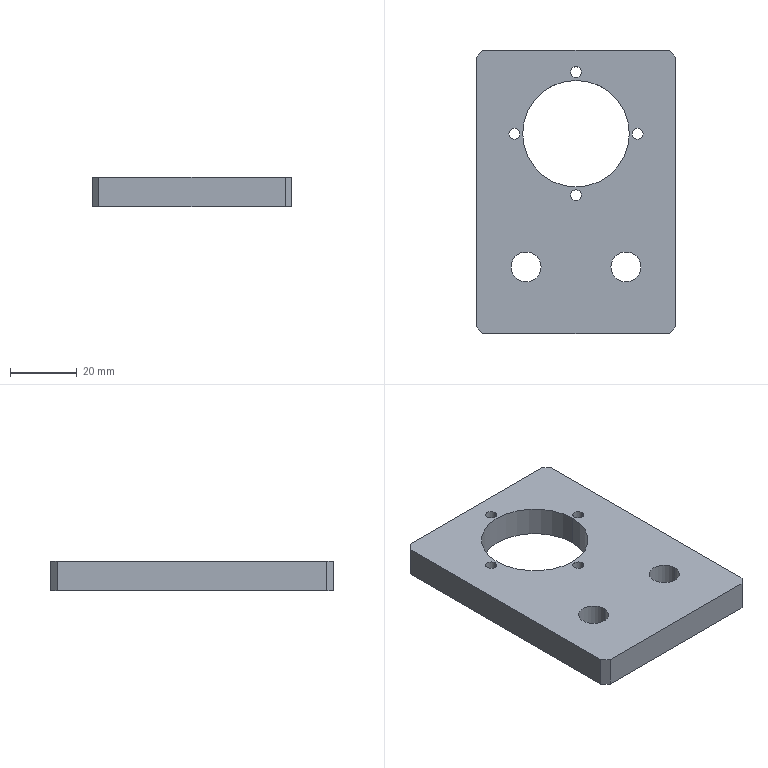Component | SolidWorks | KSD171005A-01-01-19-1 | 1 solid | 24 faces | box 60 x 85 x 9 mm | volume 37137 mm3 | cylinder 14 | plane 10 | commonest cylinder face diameters 3.3 x8 9 x4 32 x2
build123d program:
from build123d import *

# Parameters (mm, degrees)
SKETCH1_W                = 60
SKETCH1_H                = 85
BOSS_EXTRUDE1_DEPTH      = 9
SKETCH2_R                = 16
CUT_EXTRUDE1_DEPTH       = 53.794
F_9_0_9_DIAMETER_HOLE1_D = 9
M4_TAPPED_HOLE1_D        = 3.3
CIRPATTERN1_COUNT        = 4
CHAMFER1_SIZE            = 2


with BuildPart() as part:
    # Sketch1 → Boss-Extrude1 (new body)
    with BuildSketch(Plane.XY):
        Rectangle(SKETCH1_W, SKETCH1_H)
    extrude(amount=BOSS_EXTRUDE1_DEPTH)

    # Sketch2 → Cut-Extrude1 (cut, through all)
    with BuildSketch(Plane.XY.offset(9)):
        with Locations((0, 17.5)):
            Circle(SKETCH2_R)
    extrude(amount=-CUT_EXTRUDE1_DEPTH, mode=Mode.SUBTRACT)

    # 9.0 _9_ Diameter Hole1 (through all)
    with Locations(Plane.XY.offset(9)):
        with Locations((-15, -22.5), (15, -22.5)):
            Hole(F_9_0_9_DIAMETER_HOLE1_D / 2)

    # M4 Tapped Hole1 (through all)
    with Locations(Plane.XY.offset(9)):
        with Locations((0, 36)):
            m4_tapped_hole1 = Hole(M4_TAPPED_HOLE1_D / 2)

    # CirPattern1: M4 Tapped Hole1 ×4 about axis
    cirpattern1_axis = Axis((0, 17.5, 0), (0, 0, 1))
    for i in range(1, CIRPATTERN1_COUNT):
        add(m4_tapped_hole1.rotate(cirpattern1_axis, i * 360 / CIRPATTERN1_COUNT), mode=Mode.SUBTRACT)

    # Chamfer1
    chamfer1_edges = [part.edges().sort_by_distance(p)[0] for p in [
        (30, -42.5, 4.5),
        (-30, -42.5, 4.5),
        (-30, 42.5, 4.5),
        (30, 42.5, 4.5),
    ]]
    chamfer(chamfer1_edges, length=CHAMFER1_SIZE)


solid = part.part

# Placed as in the assembly
solid = solid.moved(Location((-7.111, -1.77, 348), (0, 0, 0)))
STEP:
#1=CARTESIAN_POINT('',(0.3834,0.6193,13.701));
#2=VERTEX_POINT('',#1);
#3=CARTESIAN_POINT('',(0.5133,0.6193,13.701));
#4=VERTEX_POINT('',#3);
#5=CARTESIAN_POINT('',(0.4484,0.6193,13.701));
#6=DIRECTION('',(0.,0.,1.));
#7=DIRECTION('',(1.,0.,0.));
#8=AXIS2_PLACEMENT_3D('',#5,#6,#7);
#9=CIRCLE('',#8,0.06496);
#10=EDGE_CURVE('',#2,#4,#9,.T.);
#11=ORIENTED_EDGE('',*,*,#10,.F.);
#12=CARTESIAN_POINT('',(0.3834,0.6193,14.055));
#13=VERTEX_POINT('',#12);
#14=CARTESIAN_POINT('',(0.3834,0.6193,14.055));
#15=DIRECTION('',(0.,0.,1.));
#16=VECTOR('',#15,39.37);
#17=LINE('',#14,#16);
#18=EDGE_CURVE('',#2,#13,#17,.T.);
#19=ORIENTED_EDGE('',*,*,#18,.T.);
#20=CARTESIAN_POINT('',(0.5133,0.6193,14.055));
#21=VERTEX_POINT('',#20);
#22=CARTESIAN_POINT('',(0.4484,0.6193,14.055));
#23=DIRECTION('',(0.,0.,1.));
#24=DIRECTION('',(1.,0.,0.));
#25=AXIS2_PLACEMENT_3D('',#22,#23,#24);
#26=CIRCLE('',#25,0.06496);
#27=EDGE_CURVE('',#13,#21,#26,.T.);
#28=ORIENTED_EDGE('',*,*,#27,.T.);
#29=CARTESIAN_POINT('',(0.5133,0.6193,14.055));
#30=DIRECTION('',(0.,0.,1.));
#31=VECTOR('',#30,39.37);
#32=LINE('',#29,#31);
#33=EDGE_CURVE('',#4,#21,#32,.T.);
#34=ORIENTED_EDGE('',*,*,#33,.F.);
#35=EDGE_LOOP('',(#11,#19,#28,#34));
#36=FACE_OUTER_BOUND('',#35,.T.);
#37=CARTESIAN_POINT('',(0.4484,0.6193,14.055));
#38=DIRECTION('',(0.,0.,1.));
#39=DIRECTION('',(1.,0.,0.));
#40=AXIS2_PLACEMENT_3D('',#37,#38,#39);
#41=CYLINDRICAL_SURFACE('',#40,0.06496);
#42=ADVANCED_FACE('',(#36),#41,.F.);
#43=CARTESIAN_POINT('',(-0.3449,-0.1091,13.701));
#44=VERTEX_POINT('',#43);
#45=CARTESIAN_POINT('',(-0.215,-0.1091,13.701));
#46=VERTEX_POINT('',#45);
#47=CARTESIAN_POINT('',(-0.28,-0.1091,13.701));
#48=DIRECTION('',(0.,0.,1.));
#49=DIRECTION('',(1.,0.,0.));
#50=AXIS2_PLACEMENT_3D('',#47,#48,#49);
#51=CIRCLE('',#50,0.06496);
#52=EDGE_CURVE('',#44,#46,#51,.T.);
#53=ORIENTED_EDGE('',*,*,#52,.F.);
#54=CARTESIAN_POINT('',(-0.3449,-0.1091,14.055));
#55=VERTEX_POINT('',#54);
#56=CARTESIAN_POINT('',(-0.3449,-0.1091,14.055));
#57=DIRECTION('',(0.,0.,1.));
#58=VECTOR('',#57,39.37);
#59=LINE('',#56,#58);
#60=EDGE_CURVE('',#44,#55,#59,.T.);
#61=ORIENTED_EDGE('',*,*,#60,.T.);
#62=CARTESIAN_POINT('',(-0.215,-0.1091,14.055));
#63=VERTEX_POINT('',#62);
#64=CARTESIAN_POINT('',(-0.28,-0.1091,14.055));
#65=DIRECTION('',(0.,0.,1.));
#66=DIRECTION('',(1.,0.,0.));
#67=AXIS2_PLACEMENT_3D('',#64,#65,#66);
#68=CIRCLE('',#67,0.06496);
#69=EDGE_CURVE('',#55,#63,#68,.T.);
#70=ORIENTED_EDGE('',*,*,#69,.T.);
#71=CARTESIAN_POINT('',(-0.215,-0.1091,14.055));
#72=DIRECTION('',(0.,0.,1.));
#73=VECTOR('',#72,39.37);
#74=LINE('',#71,#73);
#75=EDGE_CURVE('',#46,#63,#74,.T.);
#76=ORIENTED_EDGE('',*,*,#75,.F.);
#77=EDGE_LOOP('',(#53,#61,#70,#76));
#78=FACE_OUTER_BOUND('',#77,.T.);
#79=CARTESIAN_POINT('',(-0.28,-0.1091,14.055));
#80=DIRECTION('',(0.,0.,1.));
#81=DIRECTION('',(1.,0.,0.));
#82=AXIS2_PLACEMENT_3D('',#79,#80,#81);
#83=CYLINDRICAL_SURFACE('',#82,0.06496);
#84=ADVANCED_FACE('',(#78),#83,.F.);
#85=CARTESIAN_POINT('',(-1.073,0.6193,13.701));
#86=VERTEX_POINT('',#85);
#87=CARTESIAN_POINT('',(-0.9434,0.6193,13.701));
#88=VERTEX_POINT('',#87);
#89=CARTESIAN_POINT('',(-1.008,0.6193,13.701));
#90=DIRECTION('',(0.,0.,1.));
#91=DIRECTION('',(1.,0.,0.));
#92=AXIS2_PLACEMENT_3D('',#89,#90,#91);
#93=CIRCLE('',#92,0.06496);
#94=EDGE_CURVE('',#86,#88,#93,.T.);
#95=ORIENTED_EDGE('',*,*,#94,.F.);
#96=CARTESIAN_POINT('',(-1.073,0.6193,14.055));
#97=VERTEX_POINT('',#96);
#98=CARTESIAN_POINT('',(-1.073,0.6193,14.055));
#99=DIRECTION('',(0.,0.,1.));
#100=VECTOR('',#99,39.37);
#101=LINE('',#98,#100);
#102=EDGE_CURVE('',#86,#97,#101,.T.);
#103=ORIENTED_EDGE('',*,*,#102,.T.);
#104=CARTESIAN_POINT('',(-0.9434,0.6193,14.055));
#105=VERTEX_POINT('',#104);
#106=CARTESIAN_POINT('',(-1.008,0.6193,14.055));
#107=DIRECTION('',(0.,0.,1.));
#108=DIRECTION('',(1.,0.,0.));
#109=AXIS2_PLACEMENT_3D('',#106,#107,#108);
#110=CIRCLE('',#109,0.06496);
#111=EDGE_CURVE('',#97,#105,#110,.T.);
#112=ORIENTED_EDGE('',*,*,#111,.T.);
#113=CARTESIAN_POINT('',(-0.9434,0.6193,14.055));
#114=DIRECTION('',(0.,0.,1.));
#115=VECTOR('',#114,39.37);
#116=LINE('',#113,#115);
#117=EDGE_CURVE('',#88,#105,#116,.T.);
#118=ORIENTED_EDGE('',*,*,#117,.F.);
#119=EDGE_LOOP('',(#95,#103,#112,#118));
#120=FACE_OUTER_BOUND('',#119,.T.);
#121=CARTESIAN_POINT('',(-1.008,0.6193,14.055));
#122=DIRECTION('',(0.,0.,1.));
#123=DIRECTION('',(1.,0.,0.));
#124=AXIS2_PLACEMENT_3D('',#121,#122,#123);
#125=CYLINDRICAL_SURFACE('',#124,0.06496);
#126=ADVANCED_FACE('',(#120),#125,.F.);
#127=CARTESIAN_POINT('',(-0.3449,1.348,13.701));
#128=VERTEX_POINT('',#127);
#129=CARTESIAN_POINT('',(-0.215,1.348,13.701));
#130=VERTEX_POINT('',#129);
#131=CARTESIAN_POINT('',(-0.28,1.348,13.701));
#132=DIRECTION('',(0.,0.,1.));
#133=DIRECTION('',(1.,0.,0.));
#134=AXIS2_PLACEMENT_3D('',#131,#132,#133);
#135=CIRCLE('',#134,0.06496);
#136=EDGE_CURVE('',#128,#130,#135,.T.);
#137=ORIENTED_EDGE('',*,*,#136,.F.);
#138=CARTESIAN_POINT('',(-0.3449,1.348,14.055));
#139=VERTEX_POINT('',#138);
#140=CARTESIAN_POINT('',(-0.3449,1.348,14.055));
#141=DIRECTION('',(0.,0.,1.));
#142=VECTOR('',#141,39.37);
#143=LINE('',#140,#142);
#144=EDGE_CURVE('',#128,#139,#143,.T.);
#145=ORIENTED_EDGE('',*,*,#144,.T.);
#146=CARTESIAN_POINT('',(-0.215,1.348,14.055));
#147=VERTEX_POINT('',#146);
#148=CARTESIAN_POINT('',(-0.28,1.348,14.055));
#149=DIRECTION('',(0.,0.,1.));
#150=DIRECTION('',(1.,0.,0.));
#151=AXIS2_PLACEMENT_3D('',#148,#149,#150);
#152=CIRCLE('',#151,0.06496);
#153=EDGE_CURVE('',#139,#147,#152,.T.);
#154=ORIENTED_EDGE('',*,*,#153,.T.);
#155=CARTESIAN_POINT('',(-0.215,1.348,14.055));
#156=DIRECTION('',(0.,0.,1.));
#157=VECTOR('',#156,39.37);
#158=LINE('',#155,#157);
#159=EDGE_CURVE('',#130,#147,#158,.T.);
#160=ORIENTED_EDGE('',*,*,#159,.F.);
#161=EDGE_LOOP('',(#137,#145,#154,#160));
#162=FACE_OUTER_BOUND('',#161,.T.);
#163=CARTESIAN_POINT('',(-0.28,1.348,14.055));
#164=DIRECTION('',(0.,0.,1.));
#165=DIRECTION('',(1.,0.,0.));
#166=AXIS2_PLACEMENT_3D('',#163,#164,#165);
#167=CYLINDRICAL_SURFACE('',#166,0.06496);
#168=ADVANCED_FACE('',(#162),#167,.F.);
#169=CARTESIAN_POINT('',(-1.048,-0.9555,13.701));
#170=VERTEX_POINT('',#169);
#171=CARTESIAN_POINT('',(-0.6934,-0.9555,13.701));
#172=VERTEX_POINT('',#171);
#173=CARTESIAN_POINT('',(-0.8705,-0.9555,13.701));
#174=DIRECTION('',(0.,0.,1.));
#175=DIRECTION('',(1.,0.,0.));
#176=AXIS2_PLACEMENT_3D('',#173,#174,#175);
#177=CIRCLE('',#176,0.1772);
#178=EDGE_CURVE('',#170,#172,#177,.T.);
#179=ORIENTED_EDGE('',*,*,#178,.F.);
#180=CARTESIAN_POINT('',(-1.048,-0.9555,14.055));
#181=VERTEX_POINT('',#180);
#182=CARTESIAN_POINT('',(-1.048,-0.9555,14.055));
#183=DIRECTION('',(0.,0.,1.));
#184=VECTOR('',#183,39.37);
#185=LINE('',#182,#184);
#186=EDGE_CURVE('',#170,#181,#185,.T.);
#187=ORIENTED_EDGE('',*,*,#186,.T.);
#188=CARTESIAN_POINT('',(-0.6934,-0.9555,14.055));
#189=VERTEX_POINT('',#188);
#190=CARTESIAN_POINT('',(-0.8705,-0.9555,14.055));
#191=DIRECTION('',(0.,0.,1.));
#192=DIRECTION('',(1.,0.,0.));
#193=AXIS2_PLACEMENT_3D('',#190,#191,#192);
#194=CIRCLE('',#193,0.1772);
#195=EDGE_CURVE('',#181,#189,#194,.T.);
#196=ORIENTED_EDGE('',*,*,#195,.T.);
#197=CARTESIAN_POINT('',(-0.6934,-0.9555,14.055));
#198=DIRECTION('',(0.,0.,1.));
#199=VECTOR('',#198,39.37);
#200=LINE('',#197,#199);
#201=EDGE_CURVE('',#172,#189,#200,.T.);
#202=ORIENTED_EDGE('',*,*,#201,.F.);
#203=EDGE_LOOP('',(#179,#187,#196,#202));
#204=FACE_OUTER_BOUND('',#203,.T.);
#205=CARTESIAN_POINT('',(-0.8705,-0.9555,14.055));
#206=DIRECTION('',(0.,0.,1.));
#207=DIRECTION('',(1.,0.,0.));
#208=AXIS2_PLACEMENT_3D('',#205,#206,#207);
#209=CYLINDRICAL_SURFACE('',#208,0.1772);
#210=ADVANCED_FACE('',(#204),#209,.F.);
#211=CARTESIAN_POINT('',(0.1334,-0.9555,13.701));
#212=VERTEX_POINT('',#211);
#213=CARTESIAN_POINT('',(0.4877,-0.9555,13.701));
#214=VERTEX_POINT('',#213);
#215=CARTESIAN_POINT('',(0.3106,-0.9555,13.701));
#216=DIRECTION('',(0.,0.,1.));
#217=DIRECTION('',(1.,0.,0.));
#218=AXIS2_PLACEMENT_3D('',#215,#216,#217);
#219=CIRCLE('',#218,0.1772);
#220=EDGE_CURVE('',#212,#214,#219,.T.);
#221=ORIENTED_EDGE('',*,*,#220,.F.);
#222=CARTESIAN_POINT('',(0.1334,-0.9555,14.055));
#223=VERTEX_POINT('',#222);
#224=CARTESIAN_POINT('',(0.1334,-0.9555,14.055));
#225=DIRECTION('',(0.,0.,1.));
#226=VECTOR('',#225,39.37);
#227=LINE('',#224,#226);
#228=EDGE_CURVE('',#212,#223,#227,.T.);
#229=ORIENTED_EDGE('',*,*,#228,.T.);
#230=CARTESIAN_POINT('',(0.4877,-0.9555,14.055));
#231=VERTEX_POINT('',#230);
#232=CARTESIAN_POINT('',(0.3106,-0.9555,14.055));
#233=DIRECTION('',(0.,0.,1.));
#234=DIRECTION('',(1.,0.,0.));
#235=AXIS2_PLACEMENT_3D('',#232,#233,#234);
#236=CIRCLE('',#235,0.1772);
#237=EDGE_CURVE('',#223,#231,#236,.T.);
#238=ORIENTED_EDGE('',*,*,#237,.T.);
#239=CARTESIAN_POINT('',(0.4877,-0.9555,14.055));
#240=DIRECTION('',(0.,0.,1.));
#241=VECTOR('',#240,39.37);
#242=LINE('',#239,#241);
#243=EDGE_CURVE('',#214,#231,#242,.T.);
#244=ORIENTED_EDGE('',*,*,#243,.F.);
#245=EDGE_LOOP('',(#221,#229,#238,#244));
#246=FACE_OUTER_BOUND('',#245,.T.);
#247=CARTESIAN_POINT('',(0.3106,-0.9555,14.055));
#248=DIRECTION('',(0.,0.,1.));
#249=DIRECTION('',(1.,0.,0.));
#250=AXIS2_PLACEMENT_3D('',#247,#248,#249);
#251=CYLINDRICAL_SURFACE('',#250,0.1772);
#252=ADVANCED_FACE('',(#246),#251,.F.);
#253=CARTESIAN_POINT('',(-0.9099,0.6193,13.701));
#254=VERTEX_POINT('',#253);
#255=CARTESIAN_POINT('',(0.3499,0.6193,13.701));
#256=VERTEX_POINT('',#255);
#257=CARTESIAN_POINT('',(-0.28,0.6193,13.701));
#258=DIRECTION('',(0.,0.,1.));
#259=DIRECTION('',(1.,0.,0.));
#260=AXIS2_PLACEMENT_3D('',#257,#258,#259);
#261=CIRCLE('',#260,0.6299);
#262=EDGE_CURVE('',#254,#256,#261,.T.);
#263=ORIENTED_EDGE('',*,*,#262,.F.);
#264=CARTESIAN_POINT('',(-0.9099,0.6193,14.055));
#265=VERTEX_POINT('',#264);
#266=CARTESIAN_POINT('',(-0.9099,0.6193,13.701));
#267=DIRECTION('',(0.,0.,1.));
#268=VECTOR('',#267,39.37);
#269=LINE('',#266,#268);
#270=EDGE_CURVE('',#254,#265,#269,.T.);
#271=ORIENTED_EDGE('',*,*,#270,.T.);
#272=CARTESIAN_POINT('',(0.3499,0.6193,14.055));
#273=VERTEX_POINT('',#272);
#274=CARTESIAN_POINT('',(-0.28,0.6193,14.055));
#275=DIRECTION('',(0.,0.,1.));
#276=DIRECTION('',(1.,0.,0.));
#277=AXIS2_PLACEMENT_3D('',#274,#275,#276);
#278=CIRCLE('',#277,0.6299);
#279=EDGE_CURVE('',#265,#273,#278,.T.);
#280=ORIENTED_EDGE('',*,*,#279,.T.);
#281=CARTESIAN_POINT('',(0.3499,0.6193,13.701));
#282=DIRECTION('',(0.,0.,1.));
#283=VECTOR('',#282,39.37);
#284=LINE('',#281,#283);
#285=EDGE_CURVE('',#256,#273,#284,.T.);
#286=ORIENTED_EDGE('',*,*,#285,.F.);
#287=EDGE_LOOP('',(#263,#271,#280,#286));
#288=FACE_OUTER_BOUND('',#287,.T.);
#289=CARTESIAN_POINT('',(-0.28,0.6193,13.701));
#290=DIRECTION('',(0.,0.,1.));
#291=DIRECTION('',(1.,0.,0.));
#292=AXIS2_PLACEMENT_3D('',#289,#290,#291);
#293=CYLINDRICAL_SURFACE('',#292,0.6299);
#294=ADVANCED_FACE('',(#288),#293,.F.);
#295=CARTESIAN_POINT('',(0.9011,-1.664,13.701));
#296=VERTEX_POINT('',#295);
#297=CARTESIAN_POINT('',(0.9011,1.525,13.701));
#298=VERTEX_POINT('',#297);
#299=CARTESIAN_POINT('',(0.9011,1.604,13.701));
#300=DIRECTION('',(-0.,1.,0.));
#301=VECTOR('',#300,39.37);
#302=LINE('',#299,#301);
#303=EDGE_CURVE('',#296,#298,#302,.T.);
#304=ORIENTED_EDGE('',*,*,#303,.T.);
#305=CARTESIAN_POINT('',(0.9011,1.525,14.055));
#306=VERTEX_POINT('',#305);
#307=CARTESIAN_POINT('',(0.9011,1.525,14.055));
#308=DIRECTION('',(0.,0.,1.));
#309=VECTOR('',#308,39.37);
#310=LINE('',#307,#309);
#311=EDGE_CURVE('',#298,#306,#310,.T.);
#312=ORIENTED_EDGE('',*,*,#311,.T.);
#313=CARTESIAN_POINT('',(0.9011,-1.664,14.055));
#314=VERTEX_POINT('',#313);
#315=CARTESIAN_POINT('',(0.9011,1.604,14.055));
#316=DIRECTION('',(-0.,1.,0.));
#317=VECTOR('',#316,39.37);
#318=LINE('',#315,#317);
#319=EDGE_CURVE('',#314,#306,#318,.T.);
#320=ORIENTED_EDGE('',*,*,#319,.F.);
#321=CARTESIAN_POINT('',(0.9011,-1.664,14.055));
#322=DIRECTION('',(0.,0.,-1.));
#323=VECTOR('',#322,39.37);
#324=LINE('',#321,#323);
#325=EDGE_CURVE('',#314,#296,#324,.T.);
#326=ORIENTED_EDGE('',*,*,#325,.T.);
#327=EDGE_LOOP('',(#304,#312,#320,#326));
#328=FACE_OUTER_BOUND('',#327,.T.);
#329=CARTESIAN_POINT('',(0.9011,1.604,14.055));
#330=DIRECTION('',(-1.,-0.,0.));
#331=DIRECTION('',(0.,-1.,0.));
#332=AXIS2_PLACEMENT_3D('',#329,#330,#331);
#333=PLANE('',#332);
#334=ADVANCED_FACE('',(#328),#333,.F.);
#335=CARTESIAN_POINT('',(0.8224,1.604,13.701));
#336=VERTEX_POINT('',#335);
#337=CARTESIAN_POINT('',(-1.382,1.604,13.701));
#338=VERTEX_POINT('',#337);
#339=CARTESIAN_POINT('',(-1.461,1.604,13.701));
#340=DIRECTION('',(-1.,0.,0.));
#341=VECTOR('',#340,39.37);
#342=LINE('',#339,#341);
#343=EDGE_CURVE('',#336,#338,#342,.T.);
#344=ORIENTED_EDGE('',*,*,#343,.T.);
#345=CARTESIAN_POINT('',(-1.382,1.604,14.055));
#346=VERTEX_POINT('',#345);
#347=CARTESIAN_POINT('',(-1.382,1.604,14.055));
#348=DIRECTION('',(0.,0.,1.));
#349=VECTOR('',#348,39.37);
#350=LINE('',#347,#349);
#351=EDGE_CURVE('',#338,#346,#350,.T.);
#352=ORIENTED_EDGE('',*,*,#351,.T.);
#353=CARTESIAN_POINT('',(0.8224,1.604,14.055));
#354=VERTEX_POINT('',#353);
#355=CARTESIAN_POINT('',(-1.461,1.604,14.055));
#356=DIRECTION('',(-1.,0.,0.));
#357=VECTOR('',#356,39.37);
#358=LINE('',#355,#357);
#359=EDGE_CURVE('',#354,#346,#358,.T.);
#360=ORIENTED_EDGE('',*,*,#359,.F.);
#361=CARTESIAN_POINT('',(0.8224,1.604,14.055));
#362=DIRECTION('',(0.,0.,-1.));
#363=VECTOR('',#362,39.37);
#364=LINE('',#361,#363);
#365=EDGE_CURVE('',#354,#336,#364,.T.);
#366=ORIENTED_EDGE('',*,*,#365,.T.);
#367=EDGE_LOOP('',(#344,#352,#360,#366));
#368=FACE_OUTER_BOUND('',#367,.T.);
#369=CARTESIAN_POINT('',(-1.461,1.604,14.055));
#370=DIRECTION('',(0.,-1.,0.));
#371=DIRECTION('',(0.,0.,-1.));
#372=AXIS2_PLACEMENT_3D('',#369,#370,#371);
#373=PLANE('',#372);
#374=ADVANCED_FACE('',(#368),#373,.F.);
#375=CARTESIAN_POINT('',(-1.461,1.525,14.055));
#376=VERTEX_POINT('',#375);
#377=CARTESIAN_POINT('',(-1.461,-1.664,14.055));
#378=VERTEX_POINT('',#377);
#379=CARTESIAN_POINT('',(-1.461,1.604,14.055));
#380=DIRECTION('',(0.,-1.,0.));
#381=VECTOR('',#380,39.37);
#382=LINE('',#379,#381);
#383=EDGE_CURVE('',#376,#378,#382,.T.);
#384=ORIENTED_EDGE('',*,*,#383,.F.);
#385=CARTESIAN_POINT('',(-1.461,1.525,13.701));
#386=VERTEX_POINT('',#385);
#387=CARTESIAN_POINT('',(-1.461,1.525,14.055));
#388=DIRECTION('',(0.,0.,-1.));
#389=VECTOR('',#388,39.37);
#390=LINE('',#387,#389);
#391=EDGE_CURVE('',#376,#386,#390,.T.);
#392=ORIENTED_EDGE('',*,*,#391,.T.);
#393=CARTESIAN_POINT('',(-1.461,-1.664,13.701));
#394=VERTEX_POINT('',#393);
#395=CARTESIAN_POINT('',(-1.461,1.604,13.701));
#396=DIRECTION('',(0.,-1.,0.));
#397=VECTOR('',#396,39.37);
#398=LINE('',#395,#397);
#399=EDGE_CURVE('',#386,#394,#398,.T.);
#400=ORIENTED_EDGE('',*,*,#399,.T.);
#401=CARTESIAN_POINT('',(-1.461,-1.664,14.055));
#402=DIRECTION('',(0.,0.,1.));
#403=VECTOR('',#402,39.37);
#404=LINE('',#401,#403);
#405=EDGE_CURVE('',#394,#378,#404,.T.);
#406=ORIENTED_EDGE('',*,*,#405,.T.);
#407=EDGE_LOOP('',(#384,#392,#400,#406));
#408=FACE_OUTER_BOUND('',#407,.T.);
#409=CARTESIAN_POINT('',(-1.461,1.604,14.055));
#410=DIRECTION('',(1.,0.,0.));
#411=DIRECTION('',(-0.,1.,0.));
#412=AXIS2_PLACEMENT_3D('',#409,#410,#411);
#413=PLANE('',#412);
#414=ADVANCED_FACE('',(#408),#413,.F.);
#415=CARTESIAN_POINT('',(-1.382,-1.743,13.701));
#416=VERTEX_POINT('',#415);
#417=CARTESIAN_POINT('',(0.8224,-1.743,13.701));
#418=VERTEX_POINT('',#417);
#419=CARTESIAN_POINT('',(-1.461,-1.743,13.701));
#420=DIRECTION('',(1.,0.,0.));
#421=VECTOR('',#420,39.37);
#422=LINE('',#419,#421);
#423=EDGE_CURVE('',#416,#418,#422,.T.);
#424=ORIENTED_EDGE('',*,*,#423,.T.);
#425=CARTESIAN_POINT('',(0.8224,-1.743,14.055));
#426=VERTEX_POINT('',#425);
#427=CARTESIAN_POINT('',(0.8224,-1.743,14.055));
#428=DIRECTION('',(0.,0.,1.));
#429=VECTOR('',#428,39.37);
#430=LINE('',#427,#429);
#431=EDGE_CURVE('',#418,#426,#430,.T.);
#432=ORIENTED_EDGE('',*,*,#431,.T.);
#433=CARTESIAN_POINT('',(-1.382,-1.743,14.055));
#434=VERTEX_POINT('',#433);
#435=CARTESIAN_POINT('',(-1.461,-1.743,14.055));
#436=DIRECTION('',(1.,0.,0.));
#437=VECTOR('',#436,39.37);
#438=LINE('',#435,#437);
#439=EDGE_CURVE('',#434,#426,#438,.T.);
#440=ORIENTED_EDGE('',*,*,#439,.F.);
#441=CARTESIAN_POINT('',(-1.382,-1.743,14.055));
#442=DIRECTION('',(0.,0.,-1.));
#443=VECTOR('',#442,39.37);
#444=LINE('',#441,#443);
#445=EDGE_CURVE('',#434,#416,#444,.T.);
#446=ORIENTED_EDGE('',*,*,#445,.T.);
#447=EDGE_LOOP('',(#424,#432,#440,#446));
#448=FACE_OUTER_BOUND('',#447,.T.);
#449=CARTESIAN_POINT('',(-1.461,-1.743,14.055));
#450=DIRECTION('',(0.,1.,0.));
#451=DIRECTION('',(0.,0.,1.));
#452=AXIS2_PLACEMENT_3D('',#449,#450,#451);
#453=PLANE('',#452);
#454=ADVANCED_FACE('',(#448),#453,.F.);
#455=CARTESIAN_POINT('',(0.4484,0.6193,14.055));
#456=DIRECTION('',(0.,0.,1.));
#457=DIRECTION('',(1.,0.,0.));
#458=AXIS2_PLACEMENT_3D('',#455,#456,#457);
#459=CIRCLE('',#458,0.06496);
#460=EDGE_CURVE('',#21,#13,#459,.T.);
#461=ORIENTED_EDGE('',*,*,#460,.F.);
#462=ORIENTED_EDGE('',*,*,#27,.F.);
#463=EDGE_LOOP('',(#461,#462));
#464=FACE_BOUND('',#463,.T.);
#465=CARTESIAN_POINT('',(-0.28,-0.1091,14.055));
#466=DIRECTION('',(0.,0.,1.));
#467=DIRECTION('',(1.,0.,0.));
#468=AXIS2_PLACEMENT_3D('',#465,#466,#467);
#469=CIRCLE('',#468,0.06496);
#470=EDGE_CURVE('',#63,#55,#469,.T.);
#471=ORIENTED_EDGE('',*,*,#470,.F.);
#472=ORIENTED_EDGE('',*,*,#69,.F.);
#473=EDGE_LOOP('',(#471,#472));
#474=FACE_BOUND('',#473,.T.);
#475=CARTESIAN_POINT('',(-1.008,0.6193,14.055));
#476=DIRECTION('',(0.,0.,1.));
#477=DIRECTION('',(1.,0.,0.));
#478=AXIS2_PLACEMENT_3D('',#475,#476,#477);
#479=CIRCLE('',#478,0.06496);
#480=EDGE_CURVE('',#105,#97,#479,.T.);
#481=ORIENTED_EDGE('',*,*,#480,.F.);
#482=ORIENTED_EDGE('',*,*,#111,.F.);
#483=EDGE_LOOP('',(#481,#482));
#484=FACE_BOUND('',#483,.T.);
#485=CARTESIAN_POINT('',(-0.28,1.348,14.055));
#486=DIRECTION('',(0.,0.,1.));
#487=DIRECTION('',(1.,0.,0.));
#488=AXIS2_PLACEMENT_3D('',#485,#486,#487);
#489=CIRCLE('',#488,0.06496);
#490=EDGE_CURVE('',#147,#139,#489,.T.);
#491=ORIENTED_EDGE('',*,*,#490,.F.);
#492=ORIENTED_EDGE('',*,*,#153,.F.);
#493=EDGE_LOOP('',(#491,#492));
#494=FACE_BOUND('',#493,.T.);
#495=CARTESIAN_POINT('',(-0.8705,-0.9555,14.055));
#496=DIRECTION('',(0.,0.,1.));
#497=DIRECTION('',(1.,0.,0.));
#498=AXIS2_PLACEMENT_3D('',#495,#496,#497);
#499=CIRCLE('',#498,0.1772);
#500=EDGE_CURVE('',#189,#181,#499,.T.);
#501=ORIENTED_EDGE('',*,*,#500,.F.);
#502=ORIENTED_EDGE('',*,*,#195,.F.);
#503=EDGE_LOOP('',(#501,#502));
#504=FACE_BOUND('',#503,.T.);
#505=CARTESIAN_POINT('',(0.3106,-0.9555,14.055));
#506=DIRECTION('',(0.,0.,1.));
#507=DIRECTION('',(1.,0.,0.));
#508=AXIS2_PLACEMENT_3D('',#505,#506,#507);
#509=CIRCLE('',#508,0.1772);
#510=EDGE_CURVE('',#231,#223,#509,.T.);
#511=ORIENTED_EDGE('',*,*,#510,.F.);
#512=ORIENTED_EDGE('',*,*,#237,.F.);
#513=EDGE_LOOP('',(#511,#512));
#514=FACE_BOUND('',#513,.T.);
#515=CARTESIAN_POINT('',(-0.28,0.6193,14.055));
#516=DIRECTION('',(0.,0.,1.));
#517=DIRECTION('',(1.,0.,0.));
#518=AXIS2_PLACEMENT_3D('',#515,#516,#517);
#519=CIRCLE('',#518,0.6299);
#520=EDGE_CURVE('',#273,#265,#519,.T.);
#521=ORIENTED_EDGE('',*,*,#520,.F.);
#522=ORIENTED_EDGE('',*,*,#279,.F.);
#523=EDGE_LOOP('',(#521,#522));
#524=FACE_BOUND('',#523,.T.);
#525=ORIENTED_EDGE('',*,*,#359,.T.);
#526=CARTESIAN_POINT('',(-1.668,1.318,14.055));
#527=DIRECTION('',(-0.7071,-0.7071,0.));
#528=VECTOR('',#527,39.37);
#529=LINE('',#526,#528);
#530=EDGE_CURVE('',#346,#376,#529,.T.);
#531=ORIENTED_EDGE('',*,*,#530,.T.);
#532=ORIENTED_EDGE('',*,*,#383,.T.);
#533=CARTESIAN_POINT('',(-1.668,-1.457,14.055));
#534=DIRECTION('',(0.7071,-0.7071,0.));
#535=VECTOR('',#534,39.37);
#536=LINE('',#533,#535);
#537=EDGE_CURVE('',#378,#434,#536,.T.);
#538=ORIENTED_EDGE('',*,*,#537,.T.);
#539=ORIENTED_EDGE('',*,*,#439,.T.);
#540=CARTESIAN_POINT('',(1.108,-1.457,14.055));
#541=DIRECTION('',(0.7071,0.7071,0.));
#542=VECTOR('',#541,39.37);
#543=LINE('',#540,#542);
#544=EDGE_CURVE('',#426,#314,#543,.T.);
#545=ORIENTED_EDGE('',*,*,#544,.T.);
#546=ORIENTED_EDGE('',*,*,#319,.T.);
#547=CARTESIAN_POINT('',(1.108,1.318,14.055));
#548=DIRECTION('',(-0.7071,0.7071,0.));
#549=VECTOR('',#548,39.37);
#550=LINE('',#547,#549);
#551=EDGE_CURVE('',#306,#354,#550,.T.);
#552=ORIENTED_EDGE('',*,*,#551,.T.);
#553=EDGE_LOOP('',(#525,#531,#532,#538,#539,#545,#546,#552));
#554=FACE_OUTER_BOUND('',#553,.T.);
#555=CARTESIAN_POINT('',(-0.28,-0.0697,14.055));
#556=DIRECTION('',(0.,0.,1.));
#557=DIRECTION('',(1.,0.,0.));
#558=AXIS2_PLACEMENT_3D('',#555,#556,#557);
#559=PLANE('',#558);
#560=ADVANCED_FACE('',(#464,#474,#484,#494,#504,#514,#524,#554),#559,.T.);
#561=CARTESIAN_POINT('',(0.4484,0.6193,13.701));
#562=DIRECTION('',(0.,0.,1.));
#563=DIRECTION('',(1.,0.,0.));
#564=AXIS2_PLACEMENT_3D('',#561,#562,#563);
#565=CIRCLE('',#564,0.06496);
#566=EDGE_CURVE('',#4,#2,#565,.T.);
#567=ORIENTED_EDGE('',*,*,#566,.T.);
#568=ORIENTED_EDGE('',*,*,#10,.T.);
#569=EDGE_LOOP('',(#567,#568));
#570=FACE_BOUND('',#569,.T.);
#571=CARTESIAN_POINT('',(-0.28,-0.1091,13.701));
#572=DIRECTION('',(0.,0.,1.));
#573=DIRECTION('',(1.,0.,0.));
#574=AXIS2_PLACEMENT_3D('',#571,#572,#573);
#575=CIRCLE('',#574,0.06496);
#576=EDGE_CURVE('',#46,#44,#575,.T.);
#577=ORIENTED_EDGE('',*,*,#576,.T.);
#578=ORIENTED_EDGE('',*,*,#52,.T.);
#579=EDGE_LOOP('',(#577,#578));
#580=FACE_BOUND('',#579,.T.);
#581=CARTESIAN_POINT('',(-1.008,0.6193,13.701));
#582=DIRECTION('',(0.,0.,1.));
#583=DIRECTION('',(1.,0.,0.));
#584=AXIS2_PLACEMENT_3D('',#581,#582,#583);
#585=CIRCLE('',#584,0.06496);
#586=EDGE_CURVE('',#88,#86,#585,.T.);
#587=ORIENTED_EDGE('',*,*,#586,.T.);
#588=ORIENTED_EDGE('',*,*,#94,.T.);
#589=EDGE_LOOP('',(#587,#588));
#590=FACE_BOUND('',#589,.T.);
#591=CARTESIAN_POINT('',(-0.28,1.348,13.701));
#592=DIRECTION('',(0.,0.,1.));
#593=DIRECTION('',(1.,0.,0.));
#594=AXIS2_PLACEMENT_3D('',#591,#592,#593);
#595=CIRCLE('',#594,0.06496);
#596=EDGE_CURVE('',#130,#128,#595,.T.);
#597=ORIENTED_EDGE('',*,*,#596,.T.);
#598=ORIENTED_EDGE('',*,*,#136,.T.);
#599=EDGE_LOOP('',(#597,#598));
#600=FACE_BOUND('',#599,.T.);
#601=CARTESIAN_POINT('',(-0.8705,-0.9555,13.701));
#602=DIRECTION('',(0.,0.,1.));
#603=DIRECTION('',(1.,0.,0.));
#604=AXIS2_PLACEMENT_3D('',#601,#602,#603);
#605=CIRCLE('',#604,0.1772);
#606=EDGE_CURVE('',#172,#170,#605,.T.);
#607=ORIENTED_EDGE('',*,*,#606,.T.);
#608=ORIENTED_EDGE('',*,*,#178,.T.);
#609=EDGE_LOOP('',(#607,#608));
#610=FACE_BOUND('',#609,.T.);
#611=CARTESIAN_POINT('',(0.3106,-0.9555,13.701));
#612=DIRECTION('',(0.,0.,1.));
#613=DIRECTION('',(1.,0.,0.));
#614=AXIS2_PLACEMENT_3D('',#611,#612,#613);
#615=CIRCLE('',#614,0.1772);
#616=EDGE_CURVE('',#214,#212,#615,.T.);
#617=ORIENTED_EDGE('',*,*,#616,.T.);
#618=ORIENTED_EDGE('',*,*,#220,.T.);
#619=EDGE_LOOP('',(#617,#618));
#620=FACE_BOUND('',#619,.T.);
#621=CARTESIAN_POINT('',(-0.28,0.6193,13.701));
#622=DIRECTION('',(0.,0.,1.));
#623=DIRECTION('',(1.,0.,0.));
#624=AXIS2_PLACEMENT_3D('',#621,#622,#623);
#625=CIRCLE('',#624,0.6299);
#626=EDGE_CURVE('',#256,#254,#625,.T.);
#627=ORIENTED_EDGE('',*,*,#626,.T.);
#628=ORIENTED_EDGE('',*,*,#262,.T.);
#629=EDGE_LOOP('',(#627,#628));
#630=FACE_BOUND('',#629,.T.);
#631=ORIENTED_EDGE('',*,*,#399,.F.);
#632=CARTESIAN_POINT('',(-1.461,1.525,13.701));
#633=DIRECTION('',(0.7071,0.7071,0.));
#634=VECTOR('',#633,39.37);
#635=LINE('',#632,#634);
#636=EDGE_CURVE('',#386,#338,#635,.T.);
#637=ORIENTED_EDGE('',*,*,#636,.T.);
#638=ORIENTED_EDGE('',*,*,#343,.F.);
#639=CARTESIAN_POINT('',(0.8224,1.604,13.701));
#640=DIRECTION('',(0.7071,-0.7071,0.));
#641=VECTOR('',#640,39.37);
#642=LINE('',#639,#641);
#643=EDGE_CURVE('',#336,#298,#642,.T.);
#644=ORIENTED_EDGE('',*,*,#643,.T.);
#645=ORIENTED_EDGE('',*,*,#303,.F.);
#646=CARTESIAN_POINT('',(0.9011,-1.664,13.701));
#647=DIRECTION('',(-0.7071,-0.7071,0.));
#648=VECTOR('',#647,39.37);
#649=LINE('',#646,#648);
#650=EDGE_CURVE('',#296,#418,#649,.T.);
#651=ORIENTED_EDGE('',*,*,#650,.T.);
#652=ORIENTED_EDGE('',*,*,#423,.F.);
#653=CARTESIAN_POINT('',(-1.382,-1.743,13.701));
#654=DIRECTION('',(-0.7071,0.7071,0.));
#655=VECTOR('',#654,39.37);
#656=LINE('',#653,#655);
#657=EDGE_CURVE('',#416,#394,#656,.T.);
#658=ORIENTED_EDGE('',*,*,#657,.T.);
#659=EDGE_LOOP('',(#631,#637,#638,#644,#645,#651,#652,#658));
#660=FACE_OUTER_BOUND('',#659,.T.);
#661=CARTESIAN_POINT('',(-0.28,-0.0697,13.701));
#662=DIRECTION('',(0.,0.,1.));
#663=DIRECTION('',(1.,0.,0.));
#664=AXIS2_PLACEMENT_3D('',#661,#662,#663);
#665=PLANE('',#664);
#666=ADVANCED_FACE('',(#570,#580,#590,#600,#610,#620,#630,#660),#665,.F.);
#667=ORIENTED_EDGE('',*,*,#270,.F.);
#668=ORIENTED_EDGE('',*,*,#626,.F.);
#669=ORIENTED_EDGE('',*,*,#285,.T.);
#670=ORIENTED_EDGE('',*,*,#520,.T.);
#671=EDGE_LOOP('',(#667,#668,#669,#670));
#672=FACE_OUTER_BOUND('',#671,.T.);
#673=CARTESIAN_POINT('',(-0.28,0.6193,13.701));
#674=DIRECTION('',(0.,0.,1.));
#675=DIRECTION('',(1.,0.,0.));
#676=AXIS2_PLACEMENT_3D('',#673,#674,#675);
#677=CYLINDRICAL_SURFACE('',#676,0.6299);
#678=ADVANCED_FACE('',(#672),#677,.F.);
#679=ORIENTED_EDGE('',*,*,#228,.F.);
#680=ORIENTED_EDGE('',*,*,#616,.F.);
#681=ORIENTED_EDGE('',*,*,#243,.T.);
#682=ORIENTED_EDGE('',*,*,#510,.T.);
#683=EDGE_LOOP('',(#679,#680,#681,#682));
#684=FACE_OUTER_BOUND('',#683,.T.);
#685=CARTESIAN_POINT('',(0.3106,-0.9555,14.055));
#686=DIRECTION('',(0.,0.,1.));
#687=DIRECTION('',(1.,0.,0.));
#688=AXIS2_PLACEMENT_3D('',#685,#686,#687);
#689=CYLINDRICAL_SURFACE('',#688,0.1772);
#690=ADVANCED_FACE('',(#684),#689,.F.);
#691=ORIENTED_EDGE('',*,*,#186,.F.);
#692=ORIENTED_EDGE('',*,*,#606,.F.);
#693=ORIENTED_EDGE('',*,*,#201,.T.);
#694=ORIENTED_EDGE('',*,*,#500,.T.);
#695=EDGE_LOOP('',(#691,#692,#693,#694));
#696=FACE_OUTER_BOUND('',#695,.T.);
#697=CARTESIAN_POINT('',(-0.8705,-0.9555,14.055));
#698=DIRECTION('',(0.,0.,1.));
#699=DIRECTION('',(1.,0.,0.));
#700=AXIS2_PLACEMENT_3D('',#697,#698,#699);
#701=CYLINDRICAL_SURFACE('',#700,0.1772);
#702=ADVANCED_FACE('',(#696),#701,.F.);
#703=ORIENTED_EDGE('',*,*,#144,.F.);
#704=ORIENTED_EDGE('',*,*,#596,.F.);
#705=ORIENTED_EDGE('',*,*,#159,.T.);
#706=ORIENTED_EDGE('',*,*,#490,.T.);
#707=EDGE_LOOP('',(#703,#704,#705,#706));
#708=FACE_OUTER_BOUND('',#707,.T.);
#709=CARTESIAN_POINT('',(-0.28,1.348,14.055));
#710=DIRECTION('',(0.,0.,1.));
#711=DIRECTION('',(1.,0.,0.));
#712=AXIS2_PLACEMENT_3D('',#709,#710,#711);
#713=CYLINDRICAL_SURFACE('',#712,0.06496);
#714=ADVANCED_FACE('',(#708),#713,.F.);
#715=ORIENTED_EDGE('',*,*,#102,.F.);
#716=ORIENTED_EDGE('',*,*,#586,.F.);
#717=ORIENTED_EDGE('',*,*,#117,.T.);
#718=ORIENTED_EDGE('',*,*,#480,.T.);
#719=EDGE_LOOP('',(#715,#716,#717,#718));
#720=FACE_OUTER_BOUND('',#719,.T.);
#721=CARTESIAN_POINT('',(-1.008,0.6193,14.055));
#722=DIRECTION('',(0.,0.,1.));
#723=DIRECTION('',(1.,0.,0.));
#724=AXIS2_PLACEMENT_3D('',#721,#722,#723);
#725=CYLINDRICAL_SURFACE('',#724,0.06496);
#726=ADVANCED_FACE('',(#720),#725,.F.);
#727=ORIENTED_EDGE('',*,*,#60,.F.);
#728=ORIENTED_EDGE('',*,*,#576,.F.);
#729=ORIENTED_EDGE('',*,*,#75,.T.);
#730=ORIENTED_EDGE('',*,*,#470,.T.);
#731=EDGE_LOOP('',(#727,#728,#729,#730));
#732=FACE_OUTER_BOUND('',#731,.T.);
#733=CARTESIAN_POINT('',(-0.28,-0.1091,14.055));
#734=DIRECTION('',(0.,0.,1.));
#735=DIRECTION('',(1.,0.,0.));
#736=AXIS2_PLACEMENT_3D('',#733,#734,#735);
#737=CYLINDRICAL_SURFACE('',#736,0.06496);
#738=ADVANCED_FACE('',(#732),#737,.F.);
#739=ORIENTED_EDGE('',*,*,#18,.F.);
#740=ORIENTED_EDGE('',*,*,#566,.F.);
#741=ORIENTED_EDGE('',*,*,#33,.T.);
#742=ORIENTED_EDGE('',*,*,#460,.T.);
#743=EDGE_LOOP('',(#739,#740,#741,#742));
#744=FACE_OUTER_BOUND('',#743,.T.);
#745=CARTESIAN_POINT('',(0.4484,0.6193,14.055));
#746=DIRECTION('',(0.,0.,1.));
#747=DIRECTION('',(1.,0.,0.));
#748=AXIS2_PLACEMENT_3D('',#745,#746,#747);
#749=CYLINDRICAL_SURFACE('',#748,0.06496);
#750=ADVANCED_FACE('',(#744),#749,.F.);
#751=ORIENTED_EDGE('',*,*,#530,.F.);
#752=ORIENTED_EDGE('',*,*,#351,.F.);
#753=ORIENTED_EDGE('',*,*,#636,.F.);
#754=ORIENTED_EDGE('',*,*,#391,.F.);
#755=EDGE_LOOP('',(#751,#752,#753,#754));
#756=FACE_OUTER_BOUND('',#755,.T.);
#757=CARTESIAN_POINT('',(-1.461,1.525,14.055));
#758=DIRECTION('',(0.7071,-0.7071,0.));
#759=DIRECTION('',(0.,0.,-1.));
#760=AXIS2_PLACEMENT_3D('',#757,#758,#759);
#761=PLANE('',#760);
#762=ADVANCED_FACE('',(#756),#761,.F.);
#763=ORIENTED_EDGE('',*,*,#551,.F.);
#764=ORIENTED_EDGE('',*,*,#311,.F.);
#765=ORIENTED_EDGE('',*,*,#643,.F.);
#766=ORIENTED_EDGE('',*,*,#365,.F.);
#767=EDGE_LOOP('',(#763,#764,#765,#766));
#768=FACE_OUTER_BOUND('',#767,.T.);
#769=CARTESIAN_POINT('',(0.8224,1.604,14.055));
#770=DIRECTION('',(-0.7071,-0.7071,0.));
#771=DIRECTION('',(0.,0.,-1.));
#772=AXIS2_PLACEMENT_3D('',#769,#770,#771);
#773=PLANE('',#772);
#774=ADVANCED_FACE('',(#768),#773,.F.);
#775=ORIENTED_EDGE('',*,*,#544,.F.);
#776=ORIENTED_EDGE('',*,*,#431,.F.);
#777=ORIENTED_EDGE('',*,*,#650,.F.);
#778=ORIENTED_EDGE('',*,*,#325,.F.);
#779=EDGE_LOOP('',(#775,#776,#777,#778));
#780=FACE_OUTER_BOUND('',#779,.T.);
#781=CARTESIAN_POINT('',(0.9011,-1.664,14.055));
#782=DIRECTION('',(-0.7071,0.7071,0.));
#783=DIRECTION('',(0.,0.,-1.));
#784=AXIS2_PLACEMENT_3D('',#781,#782,#783);
#785=PLANE('',#784);
#786=ADVANCED_FACE('',(#780),#785,.F.);
#787=ORIENTED_EDGE('',*,*,#537,.F.);
#788=ORIENTED_EDGE('',*,*,#405,.F.);
#789=ORIENTED_EDGE('',*,*,#657,.F.);
#790=ORIENTED_EDGE('',*,*,#445,.F.);
#791=EDGE_LOOP('',(#787,#788,#789,#790));
#792=FACE_OUTER_BOUND('',#791,.T.);
#793=CARTESIAN_POINT('',(-1.382,-1.743,14.055));
#794=DIRECTION('',(0.7071,0.7071,0.));
#795=DIRECTION('',(0.,0.,-1.));
#796=AXIS2_PLACEMENT_3D('',#793,#794,#795);
#797=PLANE('',#796);
#798=ADVANCED_FACE('',(#792),#797,.F.);
#799=CLOSED_SHELL('',(#42,#84,#126,#168,#210,#252,#294,#334,#374,#414,#454,#560,#666,#678,#690,#702,#714,#726,#738,#750,#762,#774,#786,#798));
#800=MANIFOLD_SOLID_BREP('',#799);
#801=CARTESIAN_POINT('',(0.,0.,0.));
#802=DIRECTION('',(0.,0.,1.));
#803=DIRECTION('',(1.,0.,0.));
#804=AXIS2_PLACEMENT_3D('',#801,#802,#803);
#805=(LENGTH_UNIT()NAMED_UNIT(*)SI_UNIT($,.METRE.));
#806=LENGTH_MEASURE_WITH_UNIT(LENGTH_MEASURE(0.0254),#805);
#807=DIMENSIONAL_EXPONENTS(1.,0.,0.,0.,0.,0.,0.);
#808=(CONVERSION_BASED_UNIT('',#806)LENGTH_UNIT()NAMED_UNIT(#807));
#809=UNCERTAINTY_MEASURE_WITH_UNIT(LENGTH_MEASURE(0.00001),#808,'','');
#810=(NAMED_UNIT(*)PLANE_ANGLE_UNIT()SI_UNIT($,.RADIAN.));
#811=(NAMED_UNIT(*)SI_UNIT($,.STERADIAN.)SOLID_ANGLE_UNIT());
#812=(GEOMETRIC_REPRESENTATION_CONTEXT(3)GLOBAL_UNCERTAINTY_ASSIGNED_CONTEXT((#809))GLOBAL_UNIT_ASSIGNED_CONTEXT((#808,#810,#811))REPRESENTATION_CONTEXT('',''));
#813=ADVANCED_BREP_SHAPE_REPRESENTATION('',(#800,#804),#812);
#814=COLOUR_RGB('',0.7922,0.8196,0.9333);
#815=FILL_AREA_STYLE_COLOUR('',#814);
#816=FILL_AREA_STYLE('',(#815));
#817=SURFACE_STYLE_FILL_AREA(#816);
#818=SURFACE_SIDE_STYLE('',(#817));
#819=SURFACE_STYLE_USAGE(.BOTH.,#818);
#820=PRESENTATION_STYLE_ASSIGNMENT((#819));
#821=STYLED_ITEM('',(#820),#800);
#822=(LENGTH_UNIT()NAMED_UNIT(*)SI_UNIT($,.METRE.));
#823=LENGTH_MEASURE_WITH_UNIT(LENGTH_MEASURE(0.0254),#822);
#824=DIMENSIONAL_EXPONENTS(1.,0.,0.,0.,0.,0.,0.);
#825=(CONVERSION_BASED_UNIT('',#823)LENGTH_UNIT()NAMED_UNIT(#824));
#826=UNCERTAINTY_MEASURE_WITH_UNIT(LENGTH_MEASURE(0.00001),#825,'','');
#827=(NAMED_UNIT(*)PLANE_ANGLE_UNIT()SI_UNIT($,.RADIAN.));
#828=(NAMED_UNIT(*)SI_UNIT($,.STERADIAN.)SOLID_ANGLE_UNIT());
#829=(GEOMETRIC_REPRESENTATION_CONTEXT(3)GLOBAL_UNCERTAINTY_ASSIGNED_CONTEXT((#826))GLOBAL_UNIT_ASSIGNED_CONTEXT((#825,#827,#828))REPRESENTATION_CONTEXT('',''));
#830=MECHANICAL_DESIGN_GEOMETRIC_PRESENTATION_REPRESENTATION('',(#821),#829);
#831=PRESENTATION_LAYER_ASSIGNMENT('','',(#821));